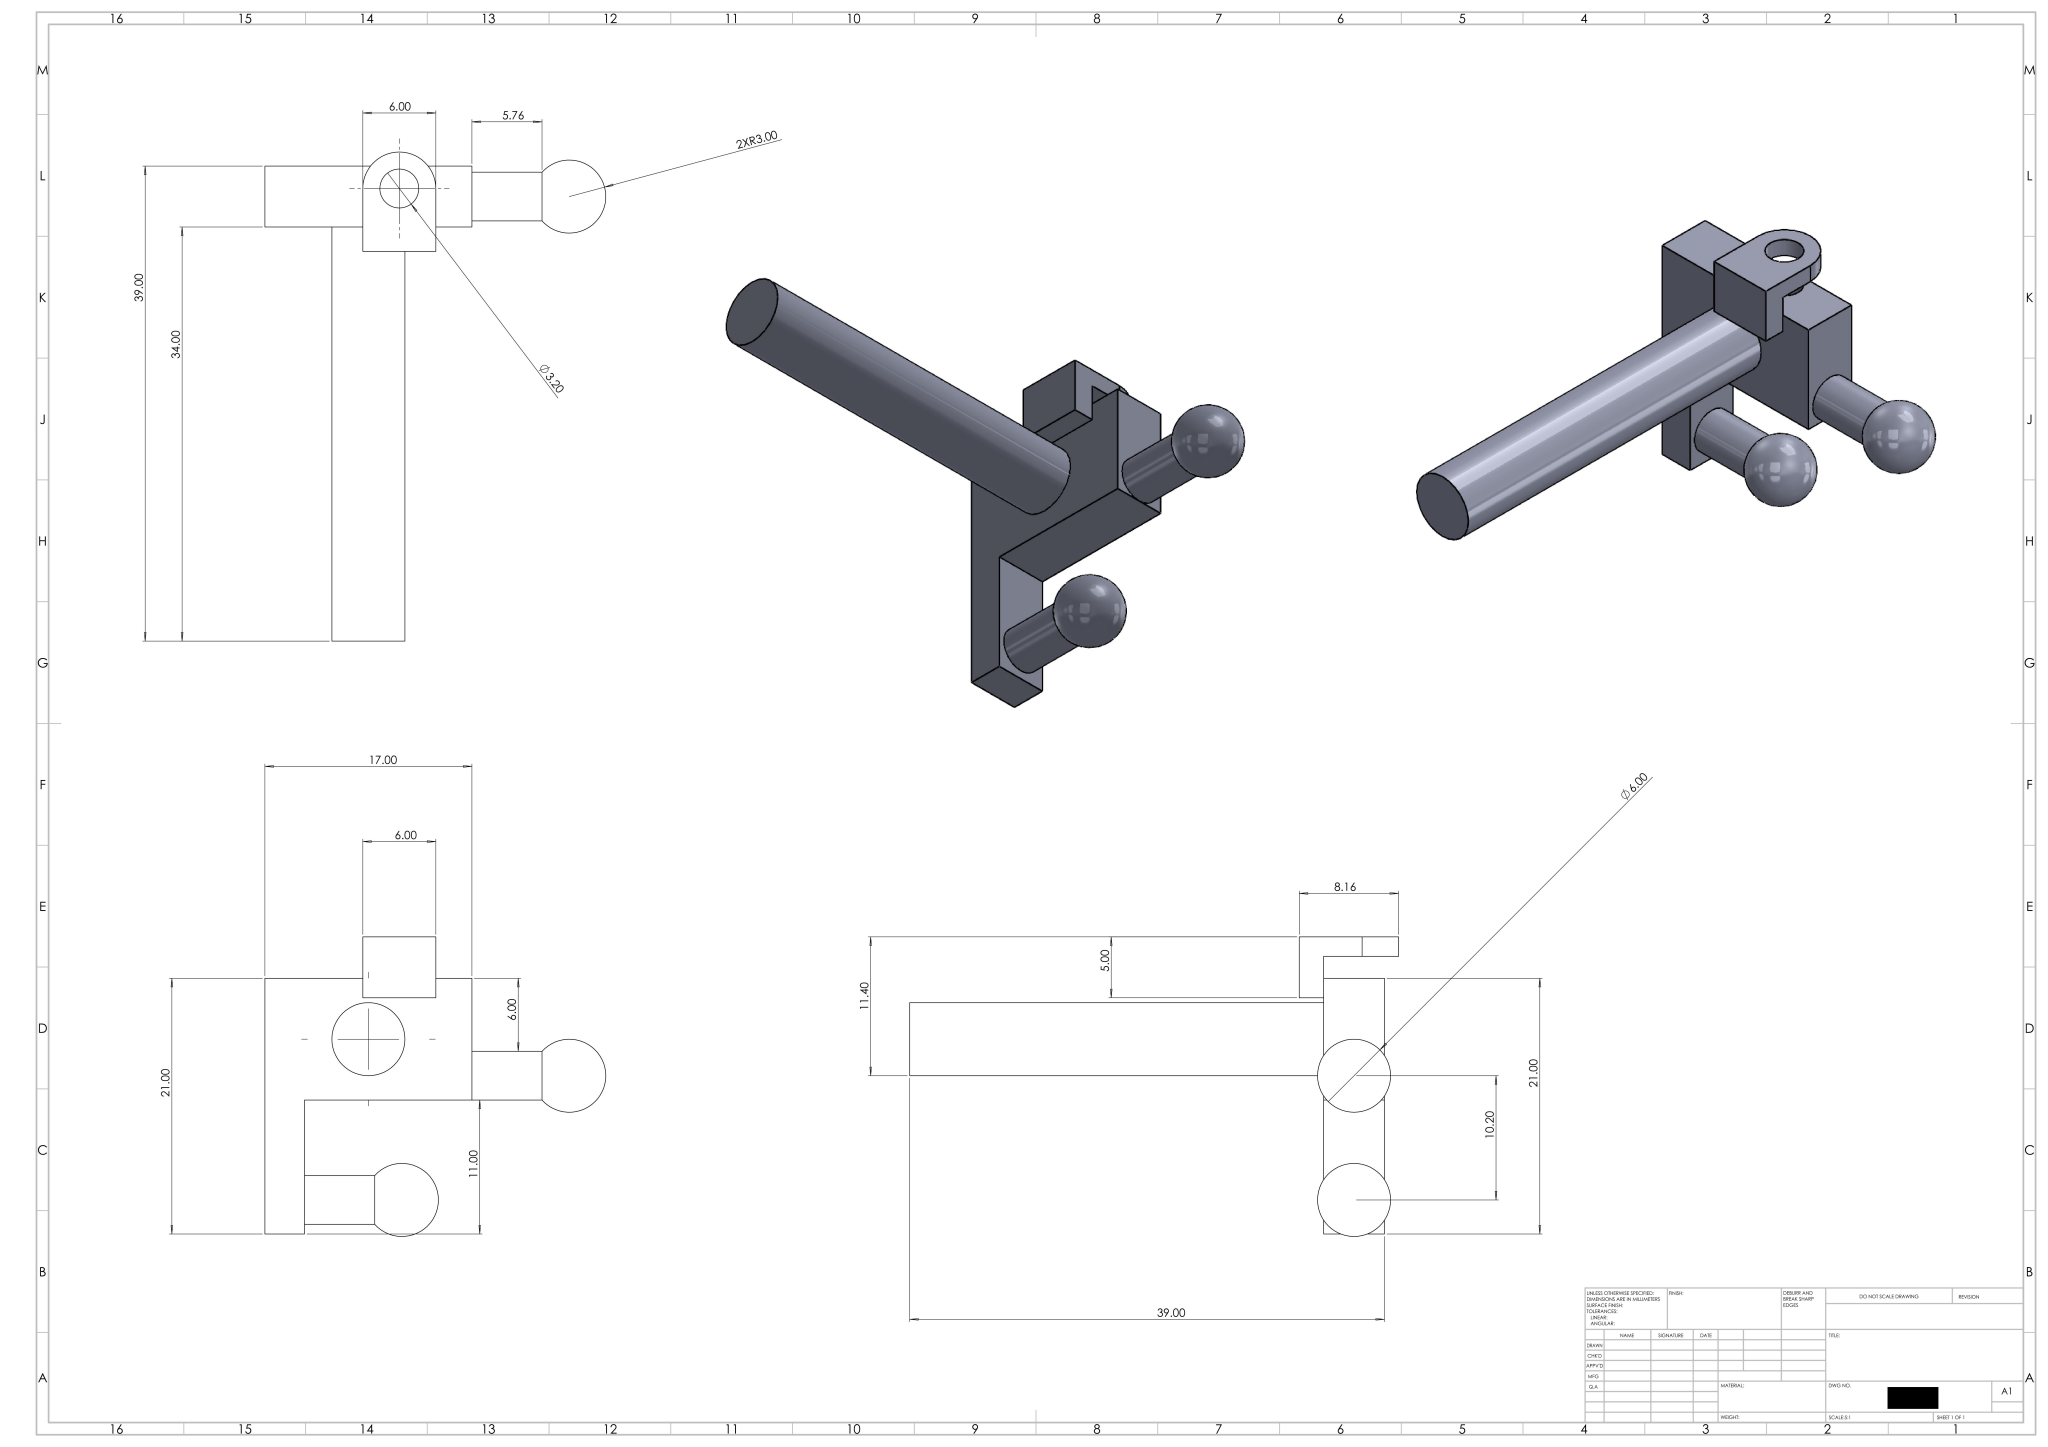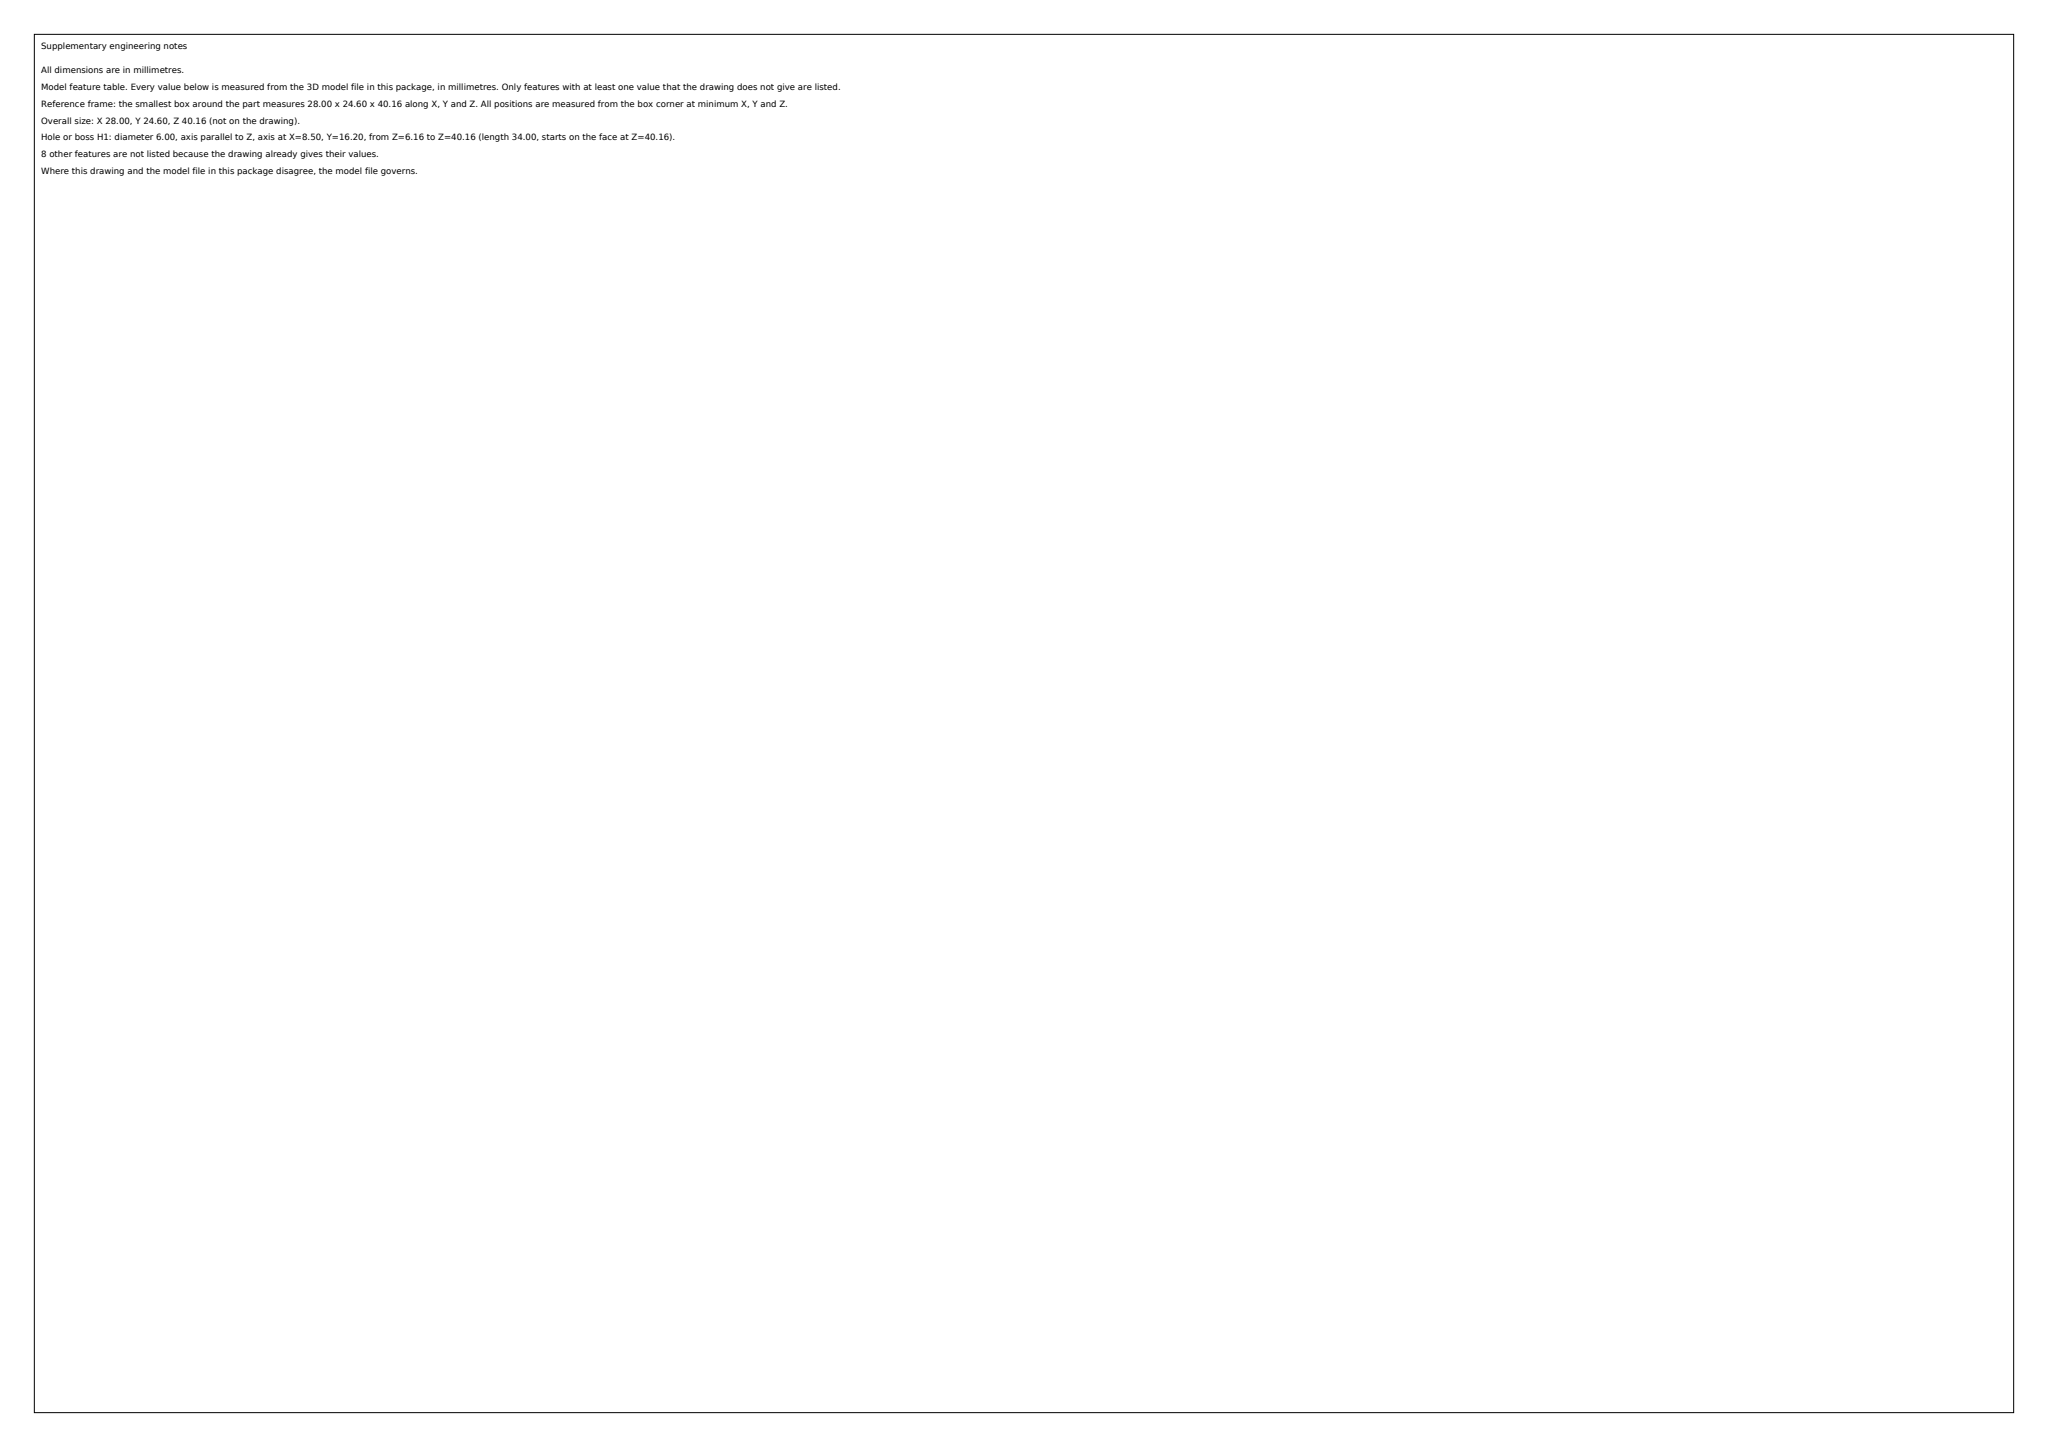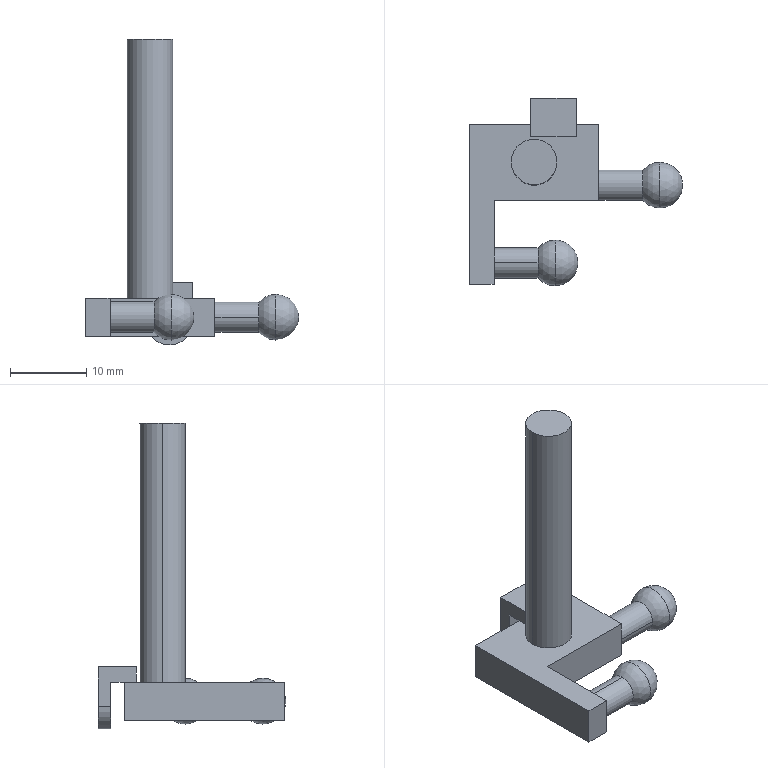Part | SolidWorks | mm | 1 solid | 32 faces | box 28 x 24.6 x 40.16 mm | volume 2431 mm3 | plane 17 | cylinder 11 | sphere 4 | commonest cylinder face diameters 3.2 x4 4 x4 6 x3
build123d program:
from build123d import *

# Parameters (mm, degrees)
SKETCH1_R           = 3
BOSS_EXTRUDE1_DEPTH = 34
BOSS_EXTRUDE2_DEPTH = 5
SKETCH3_R           = 2
BOSS_EXTRUDE3_DEPTH = 8
SKETCH5_W           = 6
SKETCH5_H           = 5
BOSS_EXTRUDE4_DEPTH = 2
SKETCH10_W          = 6
SKETCH10_H          = 1.6
BOSS_EXTRUDE6_DEPTH = 6.16
CUT_EXTRUDE2_DEPTH  = 2.1
SKETCH12_R          = 1.6
CUT_EXTRUDE3_DEPTH  = 5.85
SKETCH13_R          = 2
BOSS_EXTRUDE7_DEPTH = 8


with BuildPart() as part:
    # Sketch1 → Boss-Extrude1 (new body)
    with BuildSketch(Plane.XY):
        Circle(SKETCH1_R)
    extrude(amount=BOSS_EXTRUDE1_DEPTH)

    # Sketch2 → Boss-Extrude2 (add)
    with BuildSketch(Plane(origin=(0, 0, 0), x_dir=(-1, 0, 0), z_dir=(0, 0, -1))):
        Polygon((8.5, -5), (8.5, -16), (5.25, -16), (5.25, -5), (-8.5, -5), (-8.5, 5), (8.5, 5), align=None)
    extrude(amount=BOSS_EXTRUDE2_DEPTH)

    # Sketch3 → Boss-Extrude3 (add)
    with BuildSketch(Plane(origin=(-5.25, 0, 0), x_dir=(0, 0, -1), z_dir=(1, 0, 0))):
        with Locations(Location((2.5, -13.2, 0), (0, 0, 180))):
            Circle(SKETCH3_R)
    extrude(amount=BOSS_EXTRUDE3_DEPTH)

    # Sketch4 → Revolve1 (revolve)
    with BuildSketch(Plane(origin=(2.75, 0, 0), x_dir=(0, 0, -1), z_dir=(1, 0, 0))):
        with BuildLine():
            Line((-0.5, -13.2), (5.5, -13.2))
            ThreePointArc((5.5, -13.2), (2.5, -10.2), (-0.5, -13.2))
        make_face()
    revolve(axis=Axis((2.75, -13.2, 0.5), (0, 0, -1)))

    # Sketch5 → Boss-Extrude4 (add)
    with BuildSketch(Plane.XY):
        with Locations((2.54, 5.9)):
            Rectangle(SKETCH5_W, SKETCH5_H)
    extrude(amount=BOSS_EXTRUDE4_DEPTH)

    # Sketch10 → Boss-Extrude6 (add)
    with BuildSketch(Plane(origin=(0, 0, 0), x_dir=(-1, 0, 0), z_dir=(0, 0, -1))):
        with Locations((-2.54, 7.6)):
            Rectangle(SKETCH10_W, SKETCH10_H)
    extrude(amount=BOSS_EXTRUDE6_DEPTH)

    # Sketch11 → Cut-Extrude2 (cut)
    with BuildSketch(Plane(origin=(0, 8.4, 0), x_dir=(1, 0, 0), z_dir=(0, 1, 0))):
        with BuildLine():
            Line((-0.46, 6.16), (-0.46, 3.16))
            ThreePointArc((-0.46, 3.16), (0.4187, 5.281), (2.54, 6.16))
            Line((2.54, 6.16), (-0.46, 6.16))
        make_face()
    cut_extrude2 = extrude(amount=-CUT_EXTRUDE2_DEPTH, mode=Mode.SUBTRACT)

    # Mirror3: Cut-Extrude2 across plane
    add(cut_extrude2.mirror(Plane.ZY.offset(-2.54)), mode=Mode.SUBTRACT)

    # Sketch12 → Cut-Extrude3 (cut)
    with BuildSketch(Plane(origin=(0, 8.4, 0), x_dir=(1, 0, 0), z_dir=(0, 1, 0))):
        with Locations(Location((2.54, 3.16, 0), (0, 0, 270))):
            Circle(SKETCH12_R)
    extrude(amount=-CUT_EXTRUDE3_DEPTH, mode=Mode.SUBTRACT)

    # Sketch13 → Boss-Extrude7 (add)
    with BuildSketch(Plane(origin=(8.5, 0, 0), x_dir=(0, 0, -1), z_dir=(1, 0, 0))):
        with Locations(Location((2.5, -3, 0), (0, 0, 270))):
            Circle(SKETCH13_R)
    extrude(amount=BOSS_EXTRUDE7_DEPTH)

    # Sketch14 → Revolve2 (revolve)
    with BuildSketch(Plane(origin=(16.5, 0, 0), x_dir=(0, 0, -1), z_dir=(1, 0, 0))):
        with BuildLine():
            Line((-0.5, -3), (5.5, -3))
            ThreePointArc((5.5, -3), (2.5, 0), (-0.5, -3))
        make_face()
    revolve(axis=Axis((16.5, -3, 0.5), (0, 0, -1)))


solid = part.part